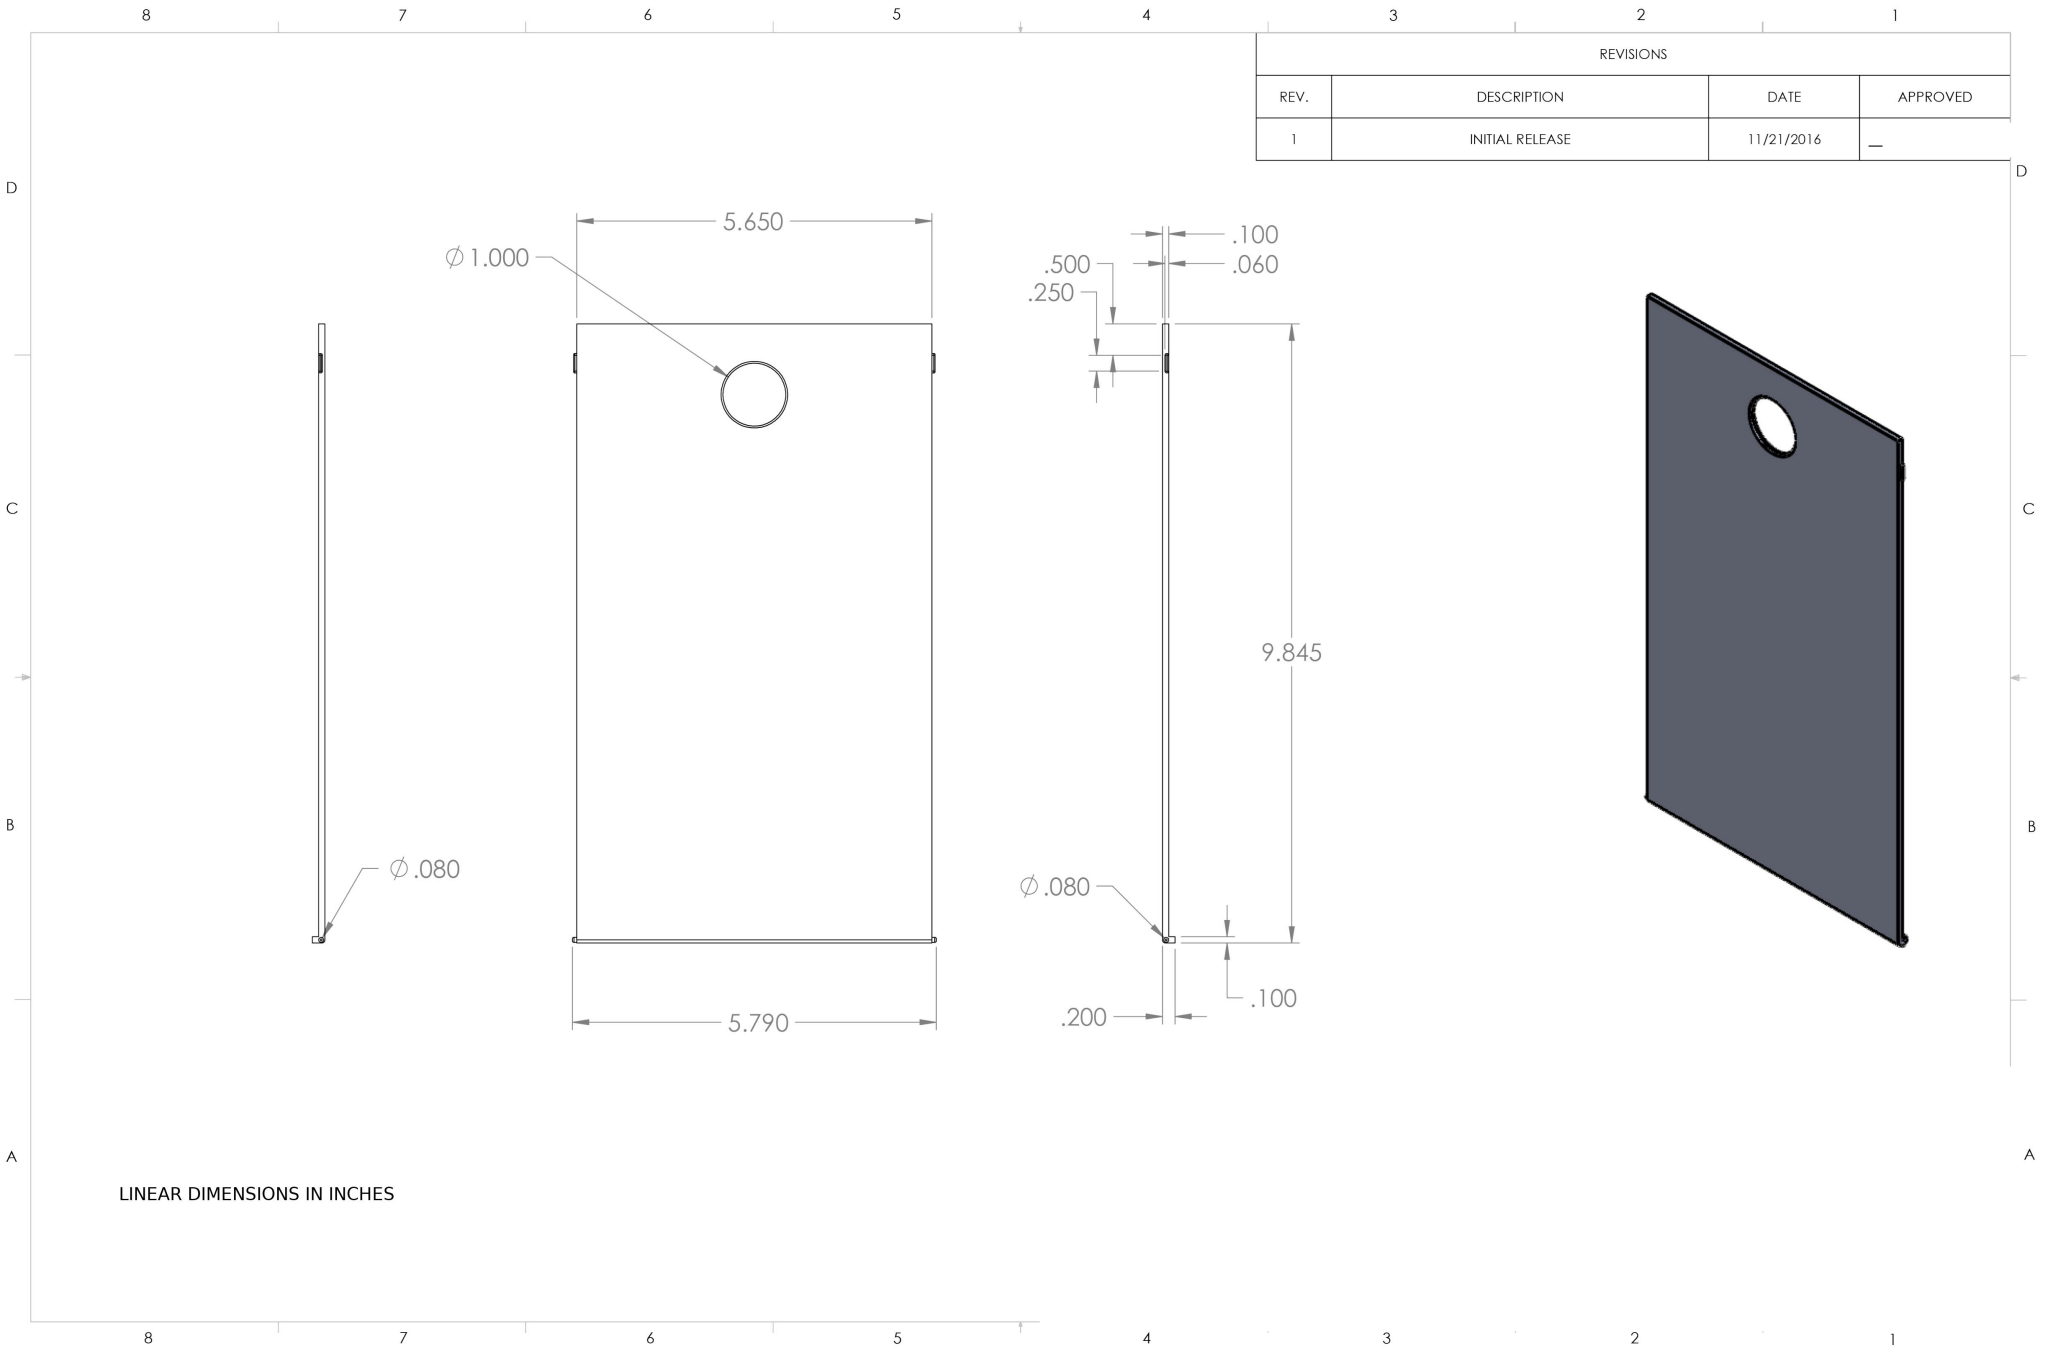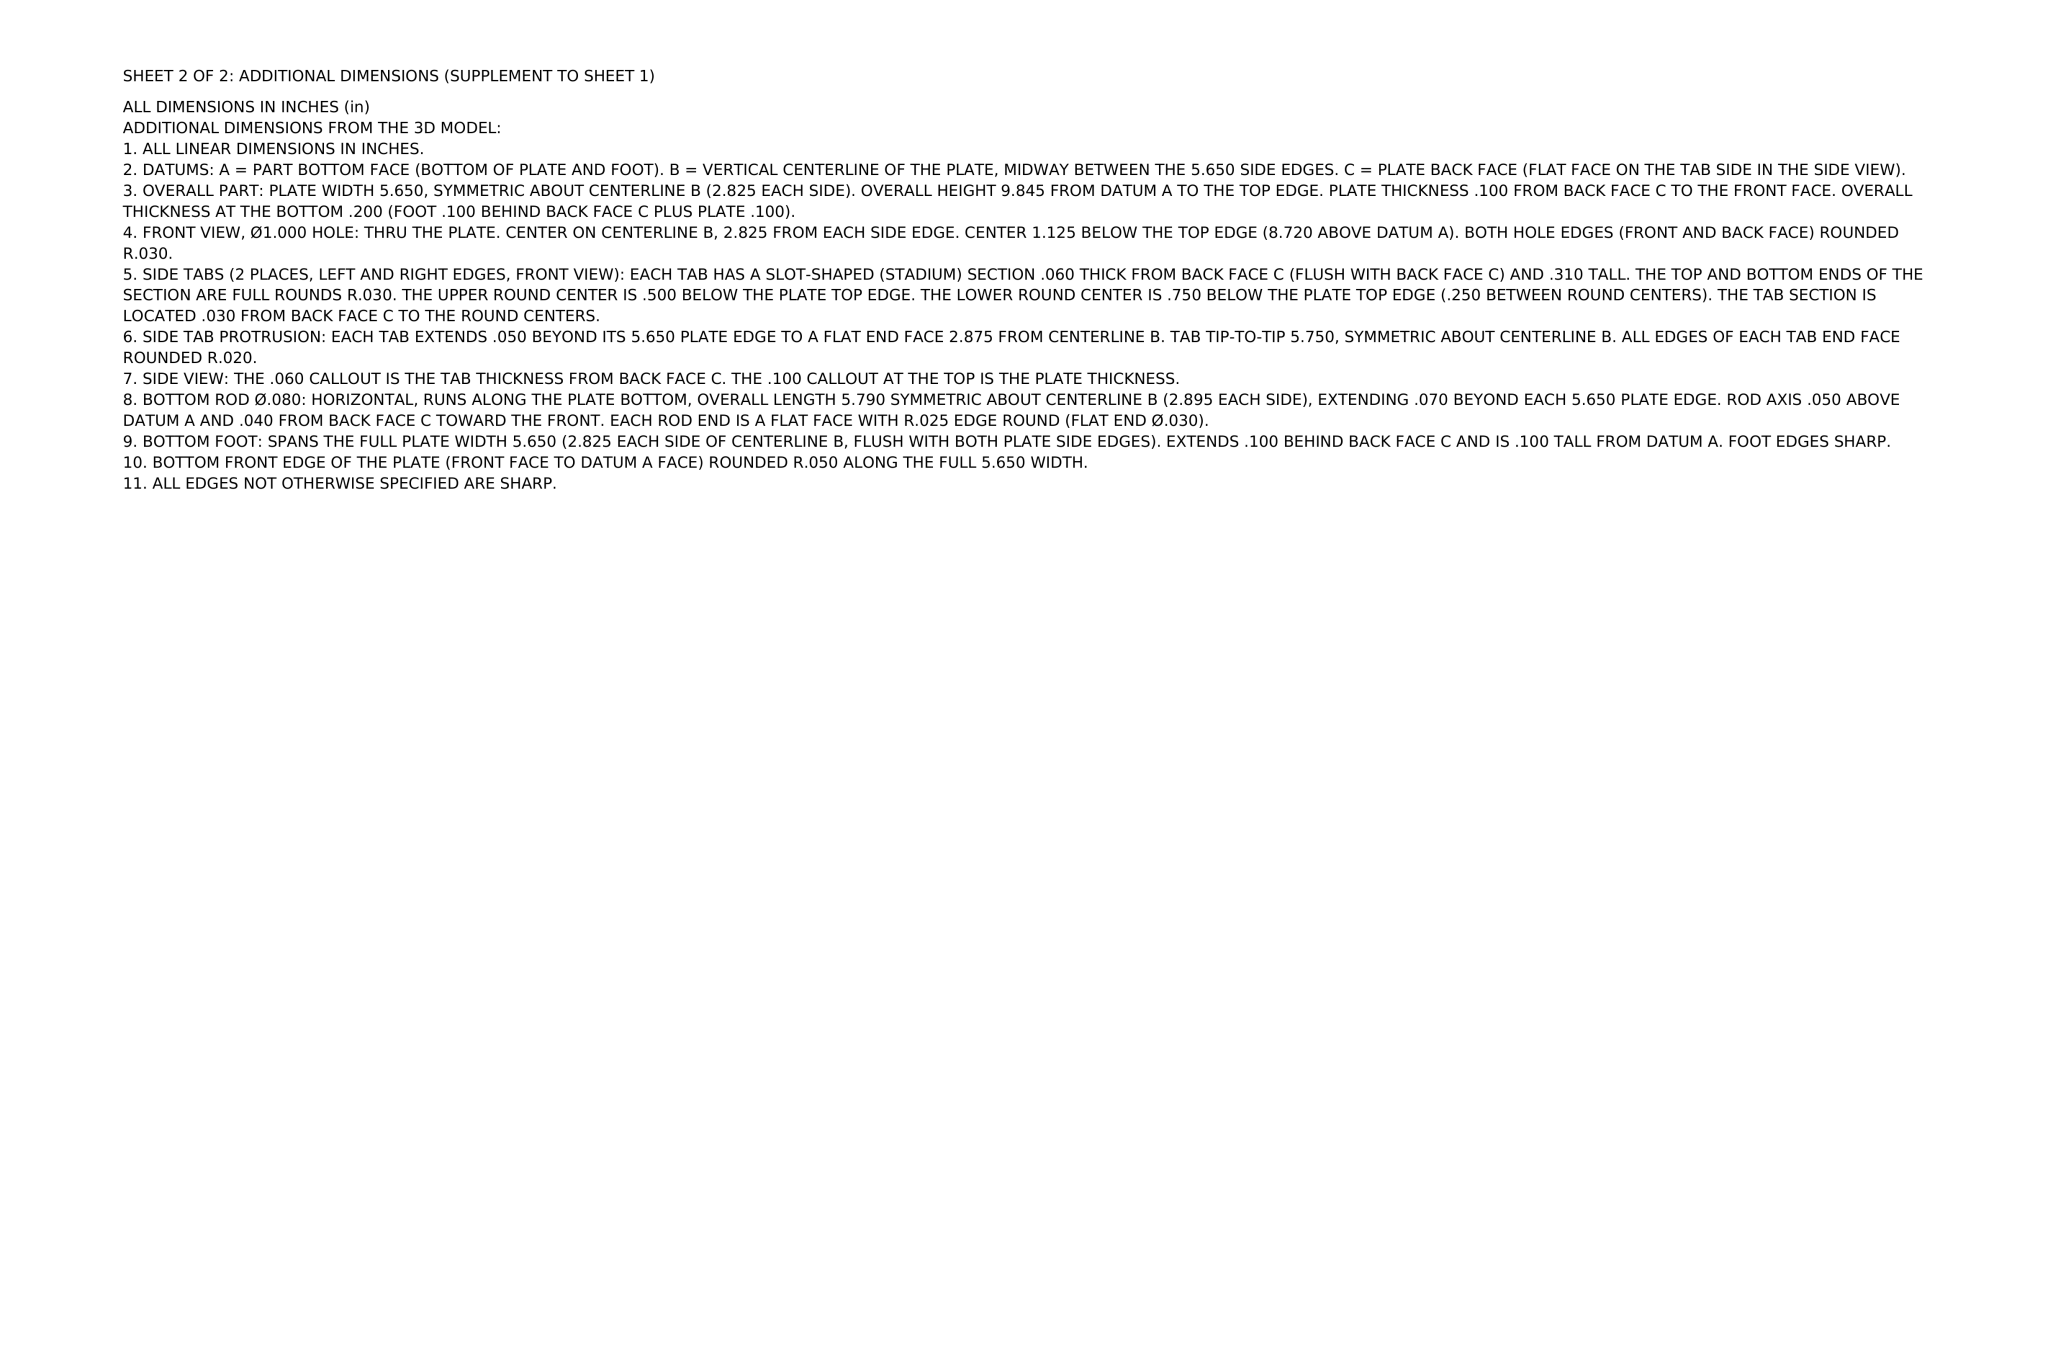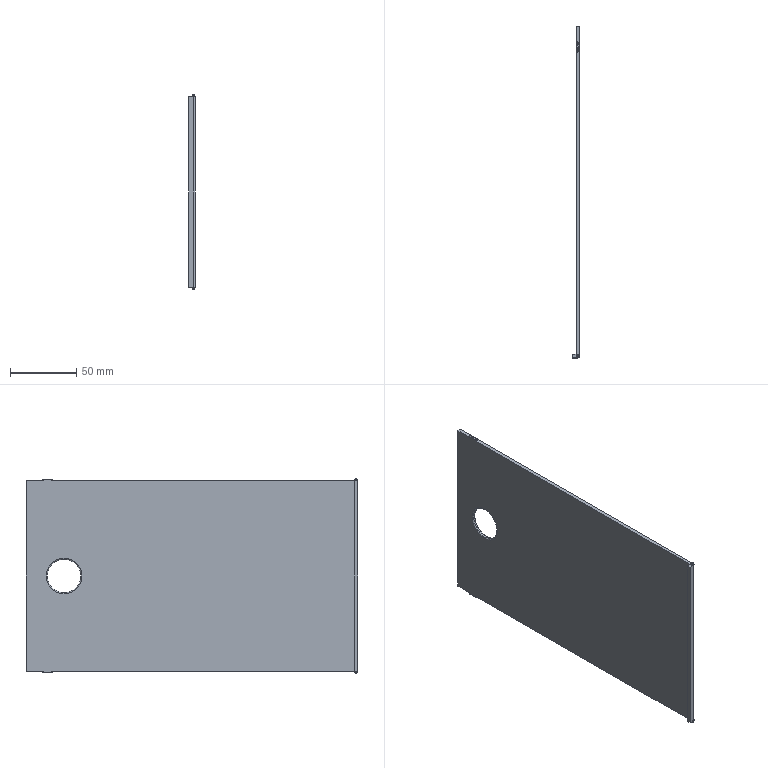Part | NX | drawing in metres | 1 solid | 41 faces | box 5.08 x 250.06 x 147.07 mm | volume 90759 mm3 | cylinder 15 | plane 14 | torus 12 | commonest cylinder face diameters 2.032 x4 1.524 x4 1.016 x4 25.4 x2 2.54 x1